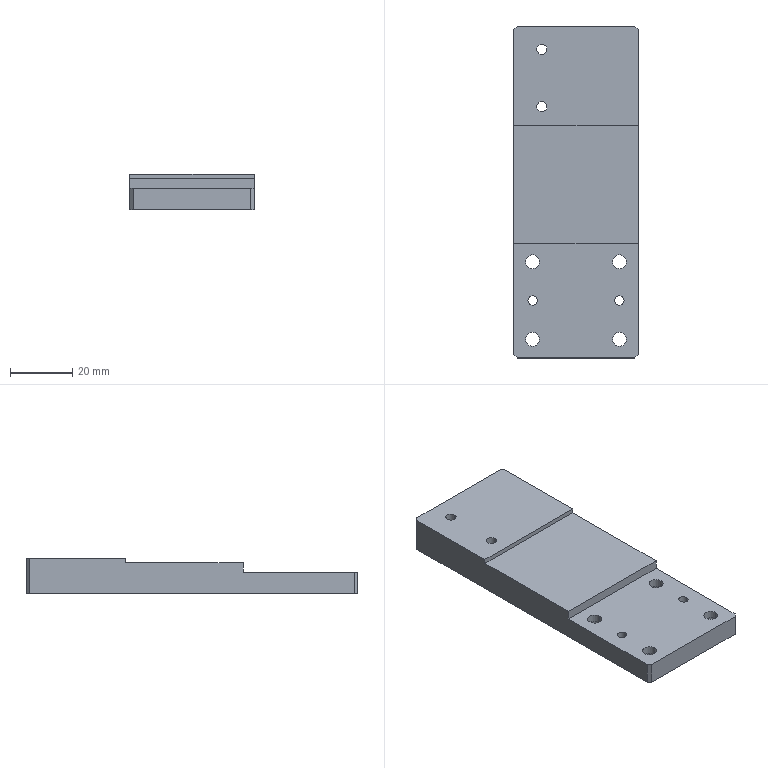Component | SolidWorks | 002MaterialPickingModuleB-1_004SidePlugModuleB-1_J-024-3 | 1 solid | 42 faces | box 40 x 107 x 11.5 mm | volume 38916 mm3 | cylinder 24 | plane 18 | commonest cylinder face diameters 8 x8 4.5 x8 3.3 x4 3 x4 | material 45
build123d program:
from build123d import *

# Parameters (mm, degrees)
SKETCH2_W                                       = 40
SKETCH2_H                                       = 107
BOSS_EXTRUDE1_DEPTH                             = 10
SKETCH3_W                                       = 40
SKETCH3_H                                       = 37
CUT_EXTRUDE1_DEPTH                              = 3
M4_HEX_SOCKET_HEAD_CAP_SCREW_CBORE1_D           = 4.5
M4_HEX_SOCKET_HEAD_CAP_SCREW_CBORE1_CBORE_D     = 8
M4_HEX_SOCKET_HEAD_CAP_SCREW_CBORE1_CBORE_DEPTH = 4.4
SIZE_MM_DOWEL_PIN_HOLE1_D                       = 3
SKETCH8_W                                       = 40
SKETCH8_H                                       = 32
BOSS_EXTRUDE2_DEPTH                             = 1.5
M4_TAPPED_HOLE1_D                               = 3.3
CHAMFER1_SIZE                                   = 1


with BuildPart() as part:
    # Sketch2 → Boss-Extrude1 (new body)
    with BuildSketch(Plane.XY):
        Rectangle(SKETCH2_W, SKETCH2_H)
    extrude(amount=BOSS_EXTRUDE1_DEPTH)

    # Sketch3 → Cut-Extrude1 (cut)
    with BuildSketch(Plane(origin=(0, 0, 0), x_dir=(-1, 0, 0), z_dir=(0, 0, -1))):
        with Locations((0, 35)):
            Rectangle(SKETCH3_W, SKETCH3_H)
    extrude(amount=-CUT_EXTRUDE1_DEPTH, mode=Mode.SUBTRACT)

    # M4 Hex Socket Head Cap Screw CBORE1 (through all)
    with Locations(Plane.XY.offset(10)):
        with Locations((-14, 47.5), (-14, 22.5), (14, 47.5), (14, 22.5)):
            CounterBoreHole(M4_HEX_SOCKET_HEAD_CAP_SCREW_CBORE1_D / 2, M4_HEX_SOCKET_HEAD_CAP_SCREW_CBORE1_CBORE_D / 2, M4_HEX_SOCKET_HEAD_CAP_SCREW_CBORE1_CBORE_DEPTH)

    # Size mm Dowel Pin Hole1 (through all)
    with Locations(Plane.XY.offset(10)):
        with Locations((-14, 35), (14, 35)):
            Hole(SIZE_MM_DOWEL_PIN_HOLE1_D / 2)

    # Sketch8 → Boss-Extrude2 (add)
    with BuildSketch(Plane(origin=(0, 0, 0), x_dir=(-1, 0, 0), z_dir=(0, 0, -1))):
        with Locations((0, -37.5)):
            Rectangle(SKETCH8_W, SKETCH8_H)
    extrude(amount=BOSS_EXTRUDE2_DEPTH)

    # M4 Tapped Hole1 (through all)
    with Locations(Plane(origin=(0, 0, -1.5), x_dir=(-1, 0, 0), z_dir=(0, 0, -1))):
        with Locations((11, -27.5), (11, -46)):
            Hole(M4_TAPPED_HOLE1_D / 2)

    # Chamfer1
    chamfer1_edges = [part.edges().sort_by_distance(p)[0] for p in [
        (-20, 53.5, 6.5),
        (20, 53.5, 6.5),
        (20, -53.5, 4.25),
        (-20, -53.5, 4.25),
    ]]
    chamfer(chamfer1_edges, length=CHAMFER1_SIZE)


solid = part.part

# Placed as in the assembly
solid = solid.moved(Location((220.325, 344.519, 63.731), (180, 0, 0)))